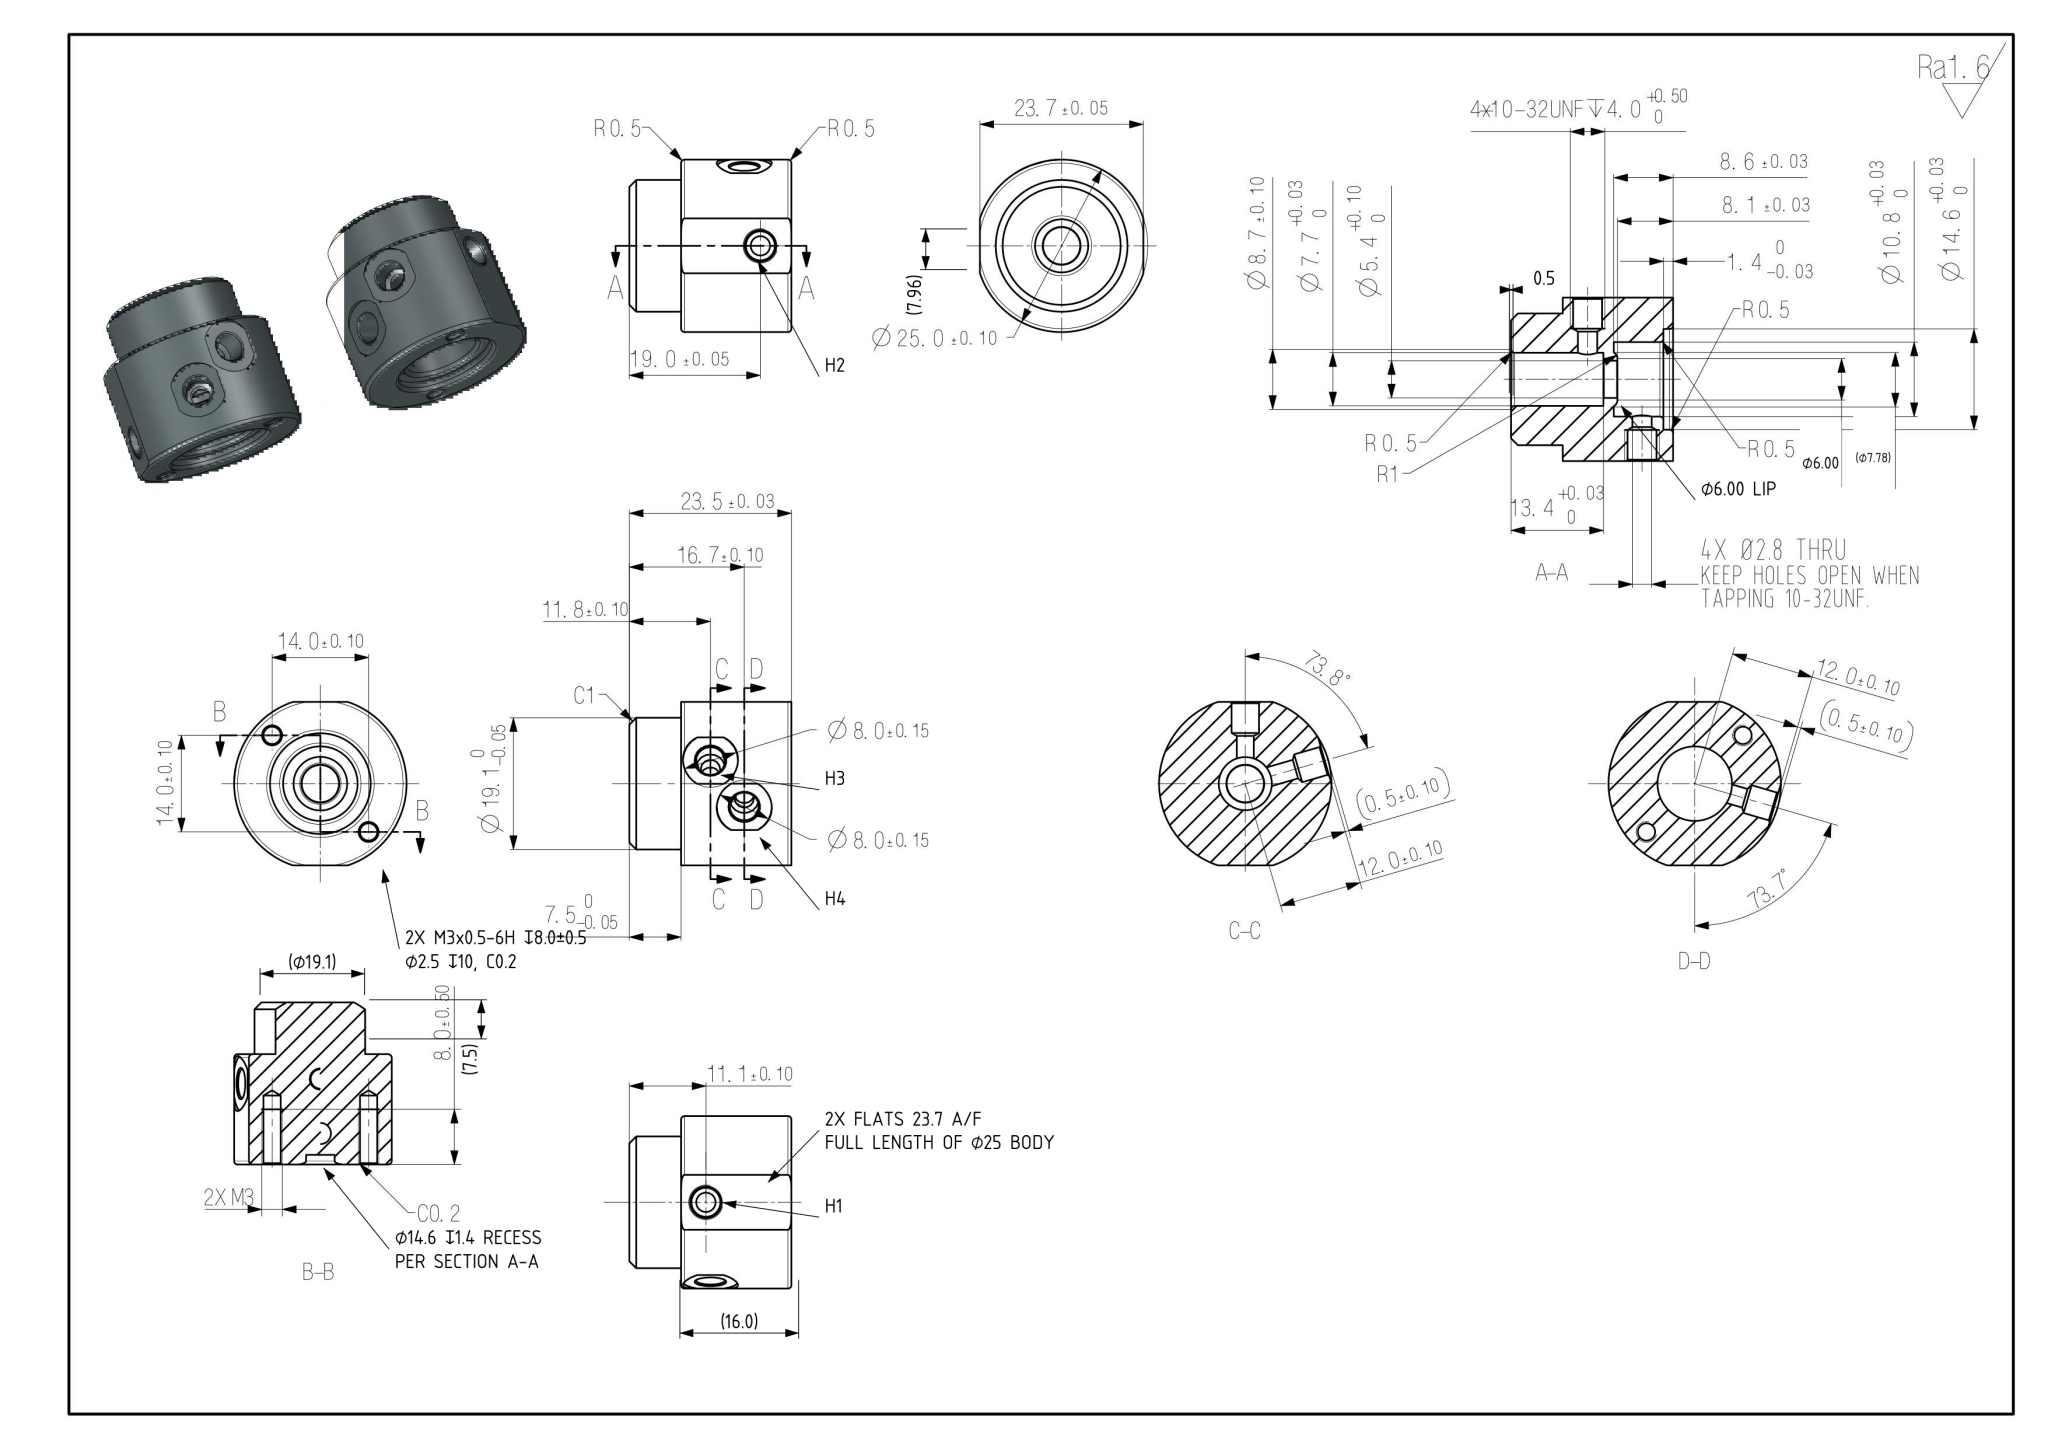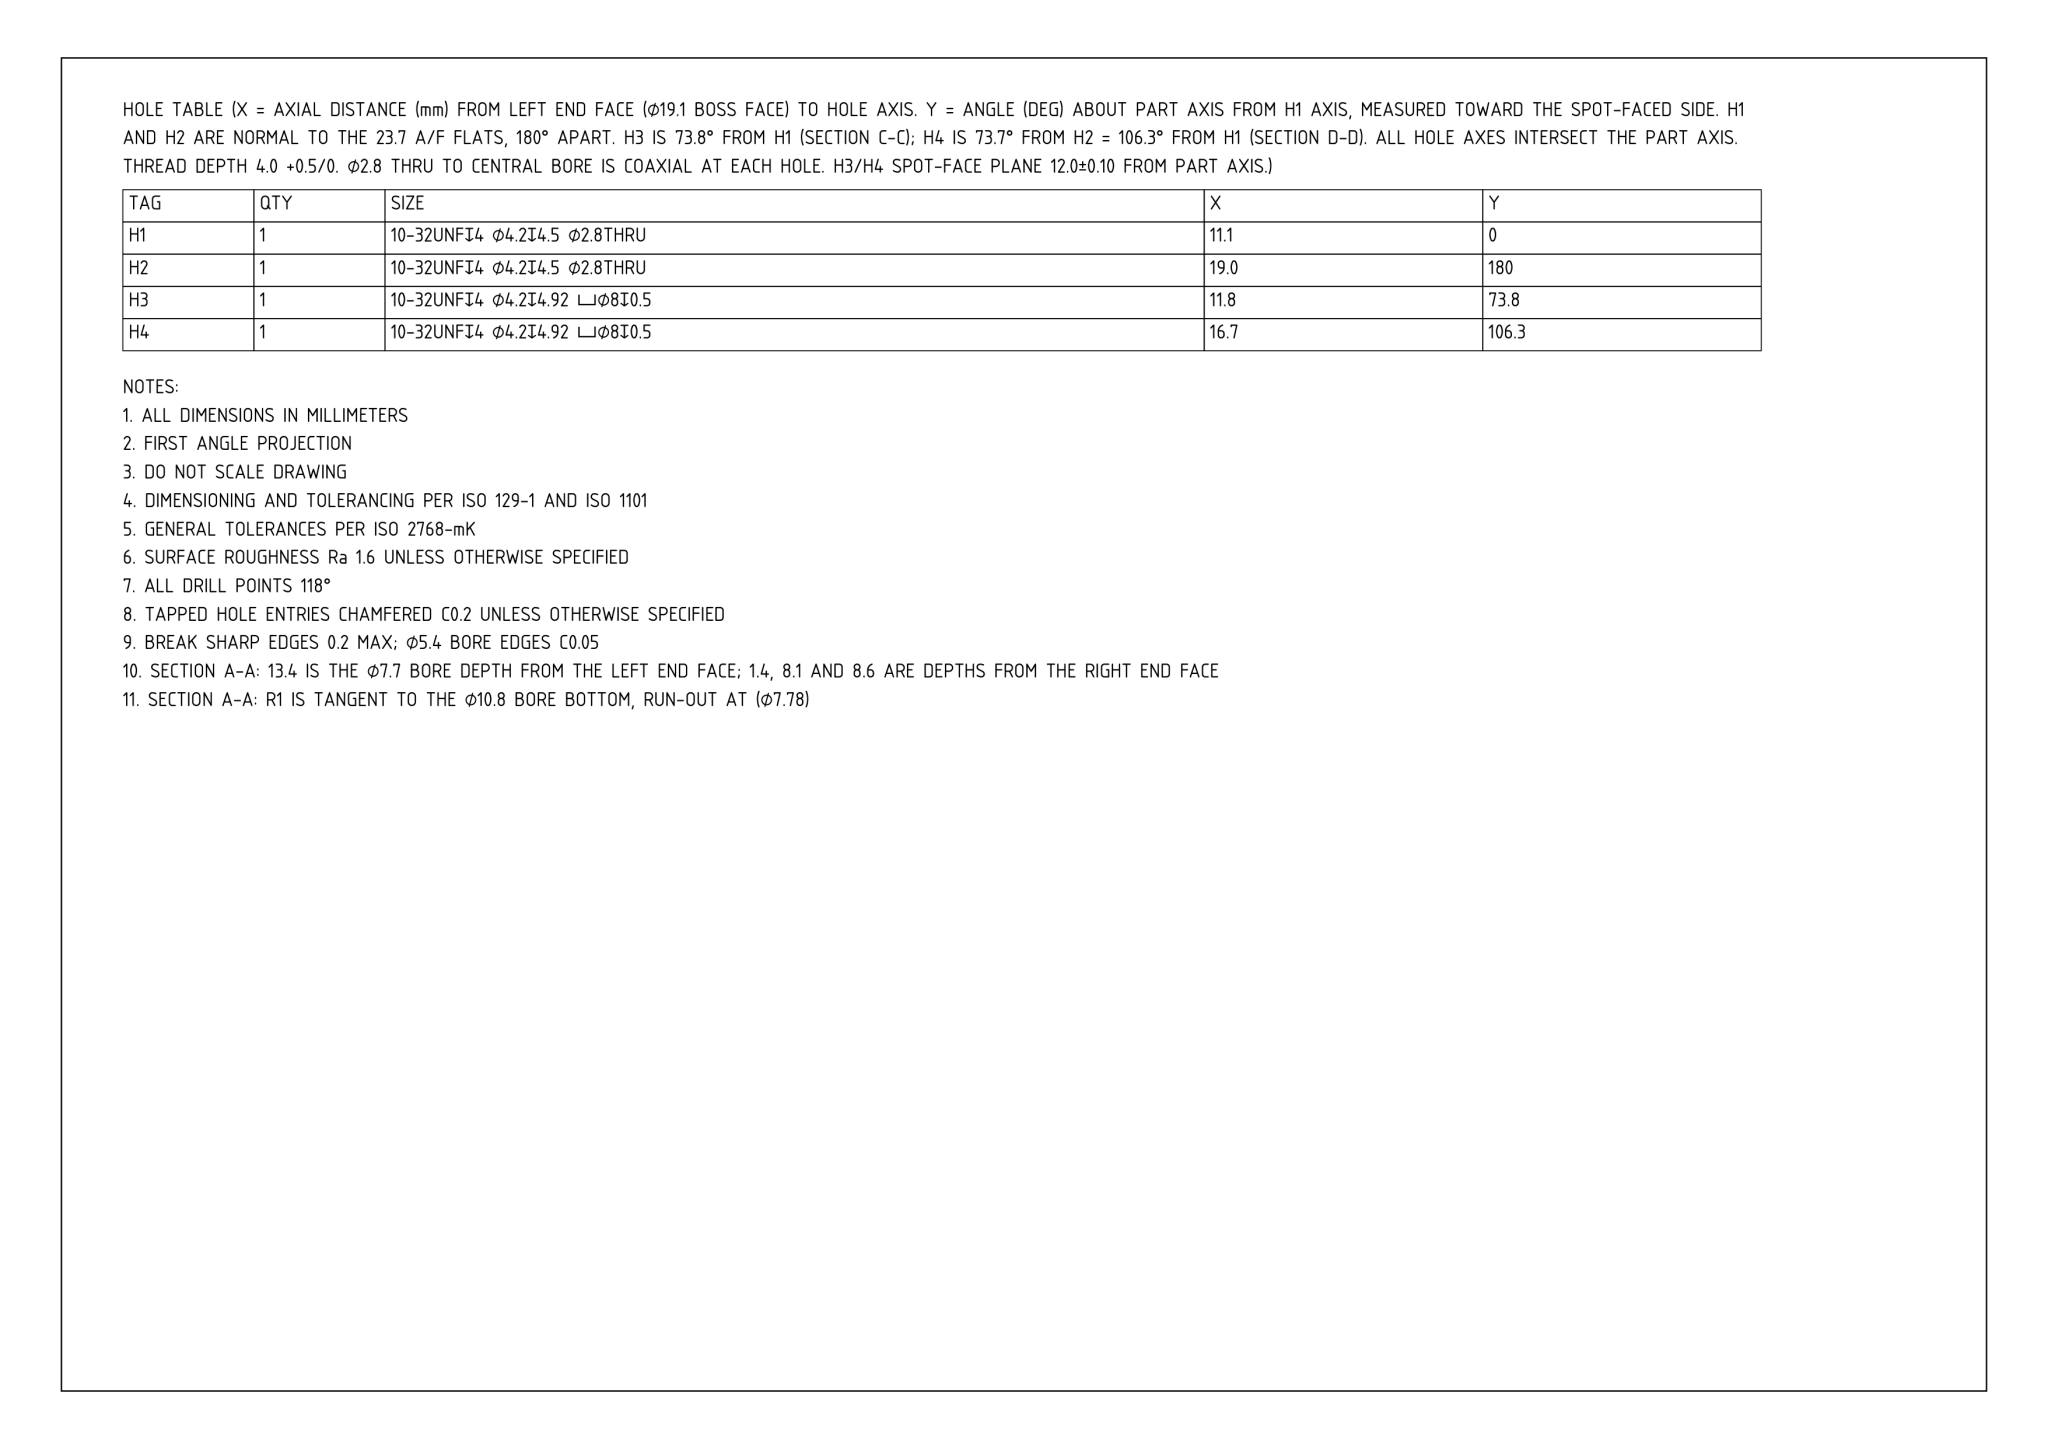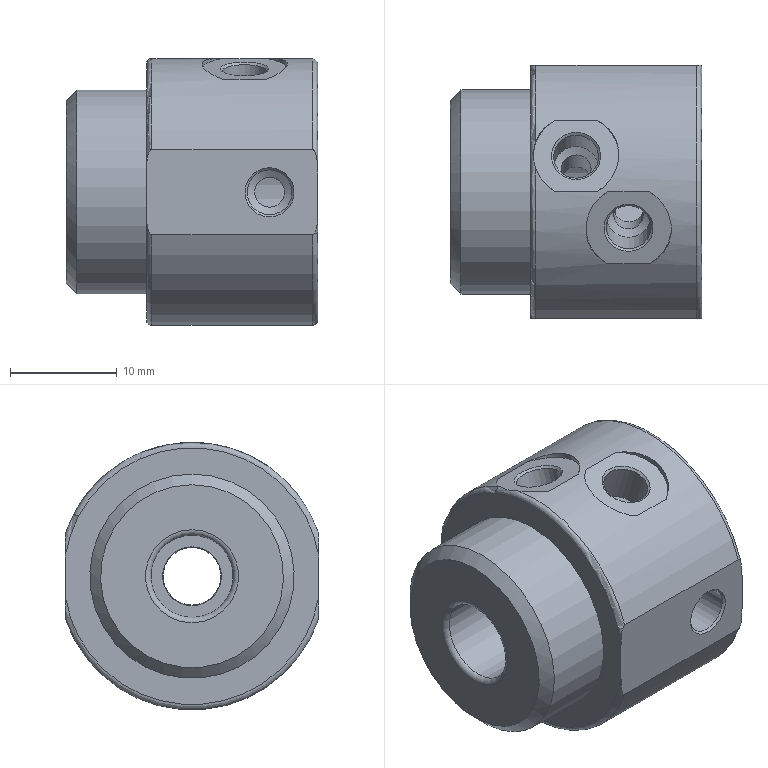Part | NX | mm | 1 solid | 55 faces | box 23.5 x 23.7 x 25 mm | volume 7854 mm3 | cylinder 21 | cone 15 | plane 11 | torus 8 | commonest cylinder face diameters 2.8 x4 4.2 x4 8 x4 25 x2 2.5 x2 19.1 x1 14.6 x1 10.8 x1